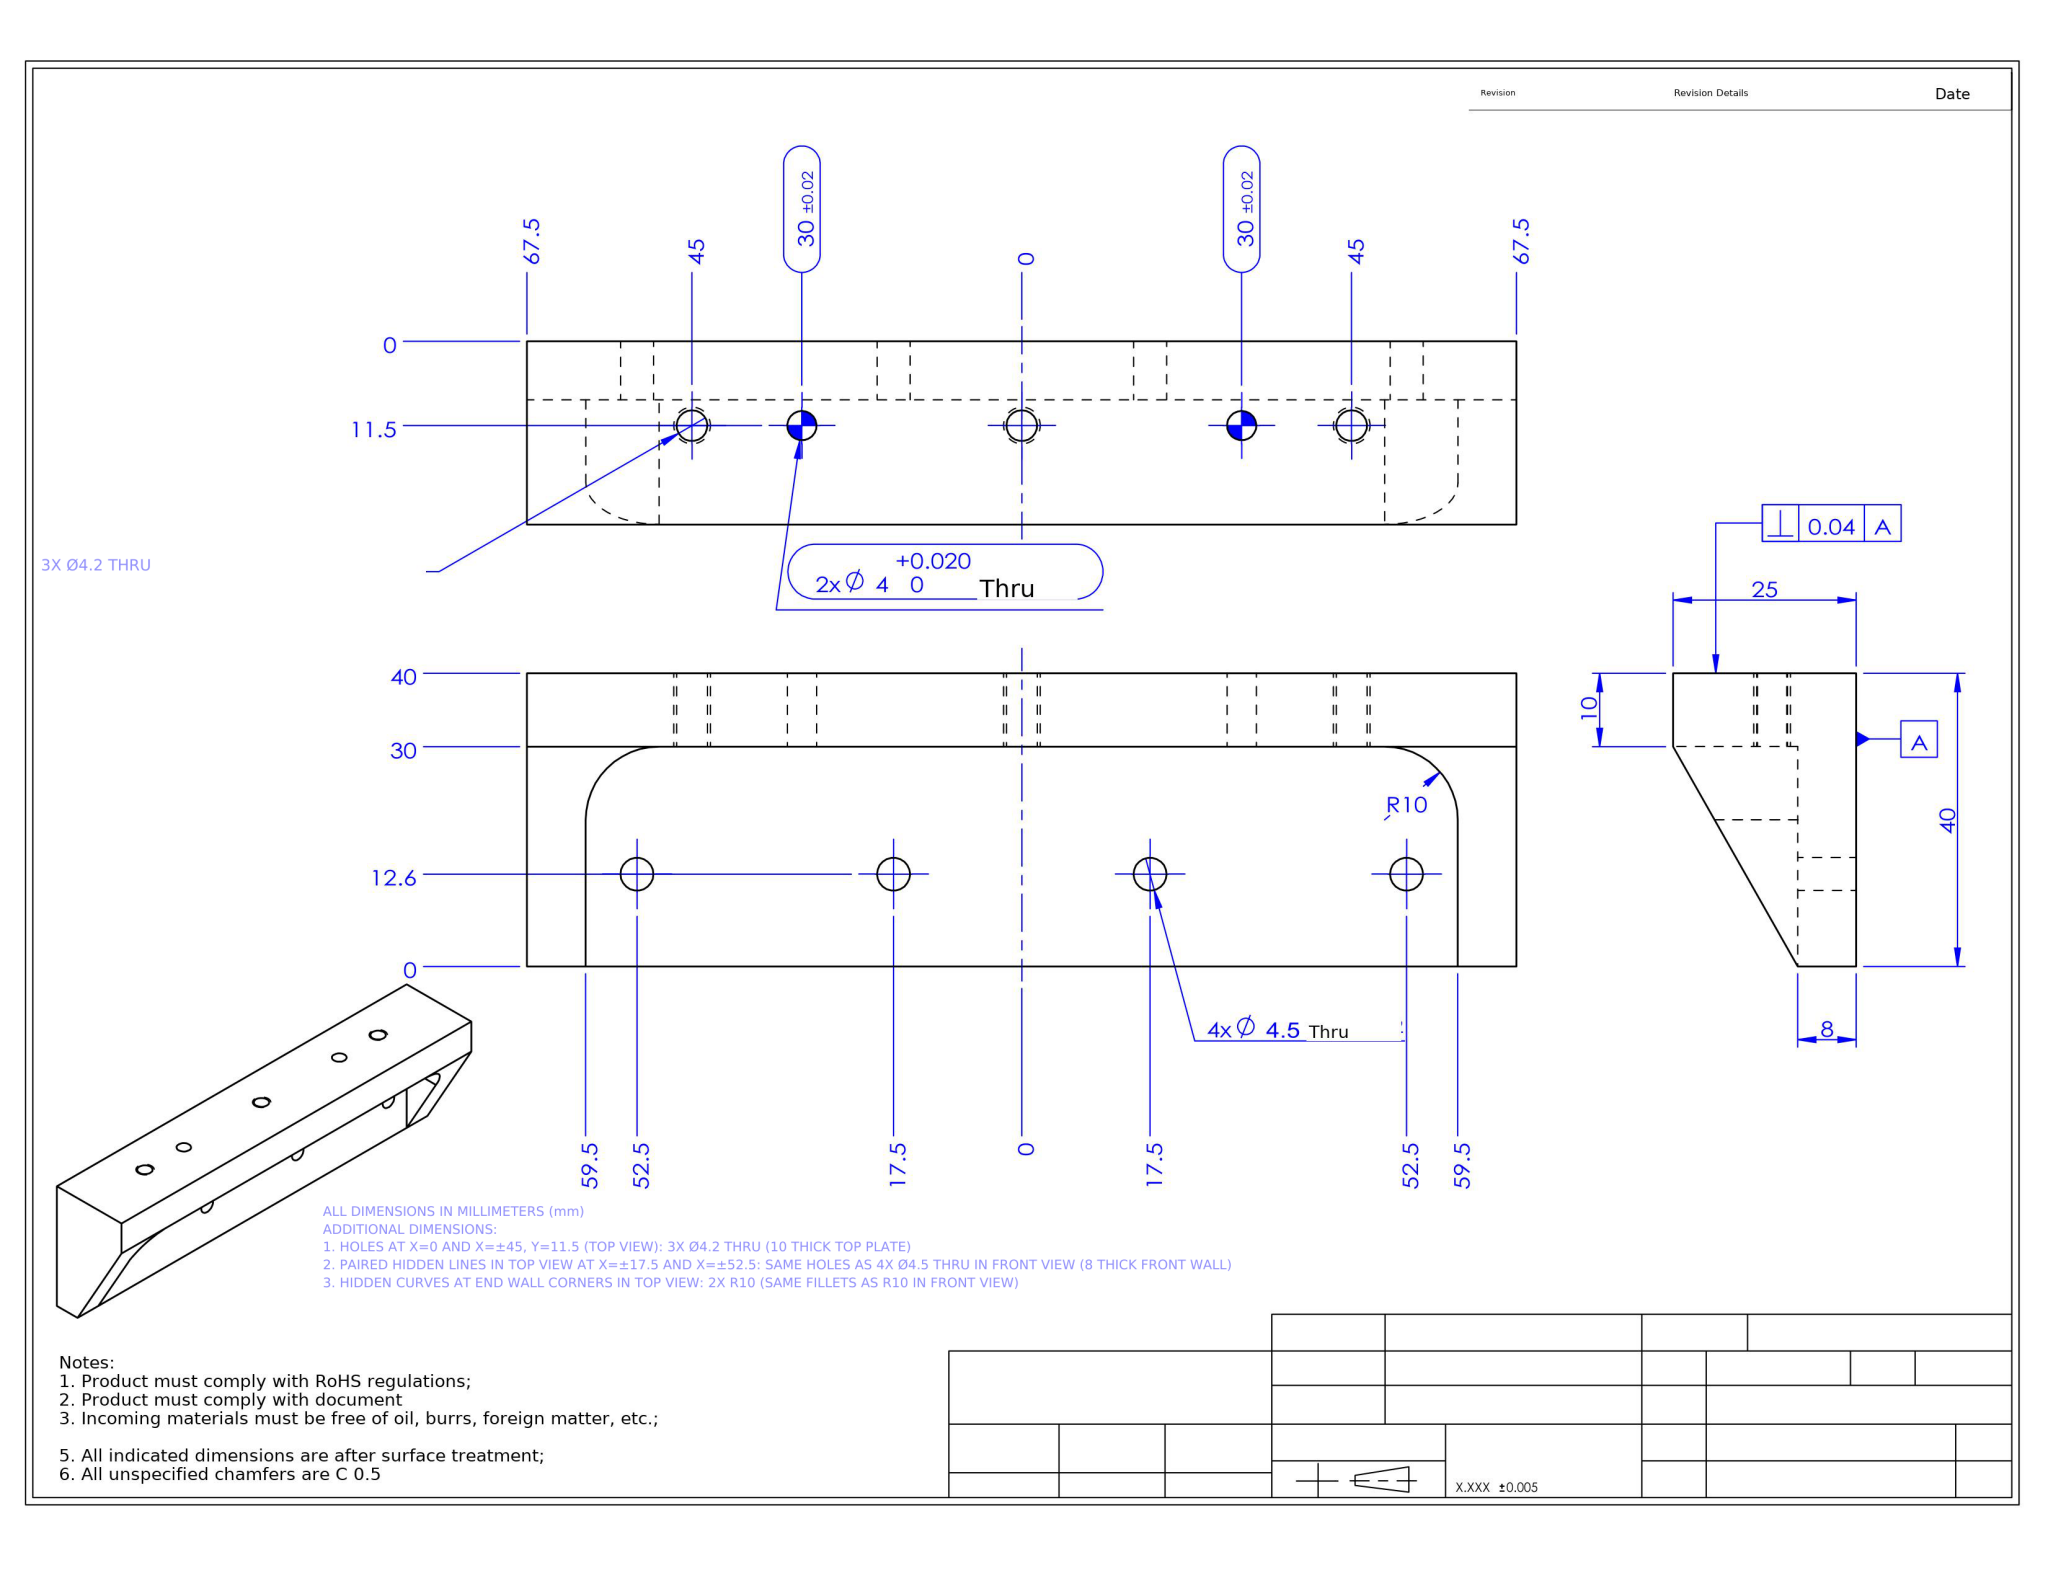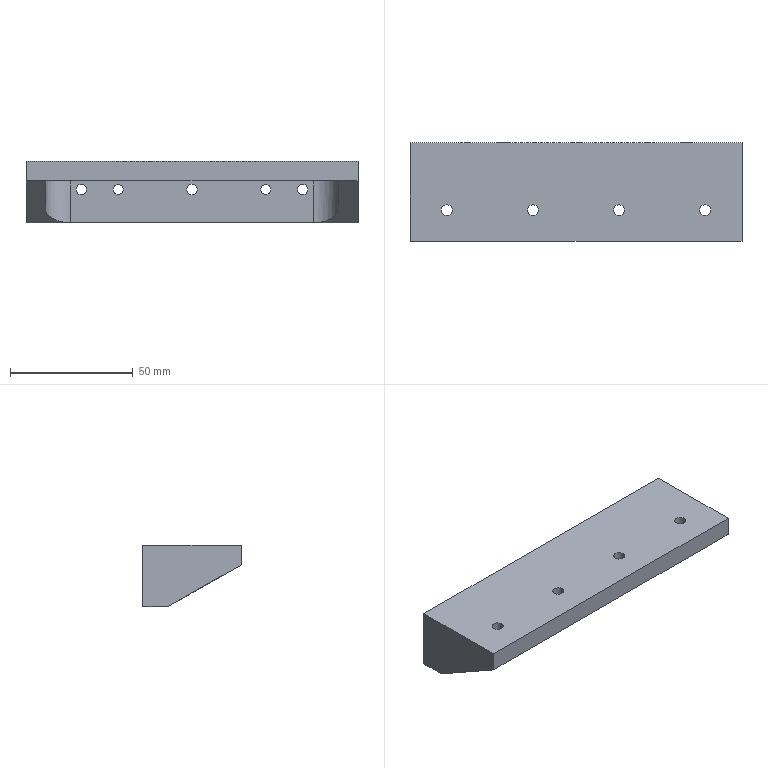Part | NX | mm | 1 solid | 32 faces | box 135 x 40 x 25 mm | volume 69729 mm3 | cylinder 20 | plane 12 | commonest cylinder face diameters 4.5 x8 4.2 x6 4 x4 20 x2